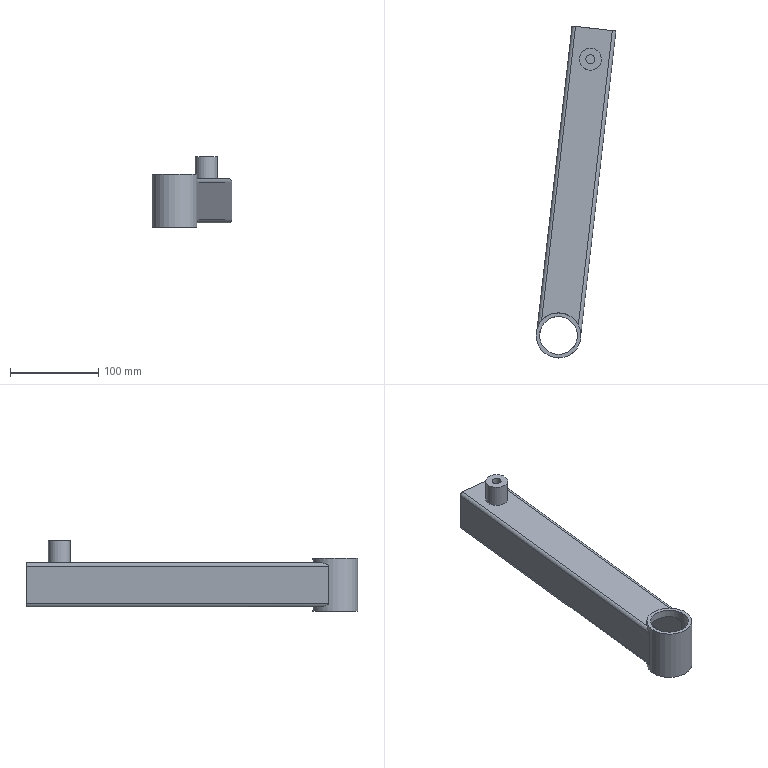Component | NX | ADJ_ROD_OUT_FRAME | 1 solid | 25 faces | volume 282819 mm3 | plane 13 | cylinder 12 | commonest cylinder face diameters 8 x8 51 x1 43 x1 25 x1 10 x1